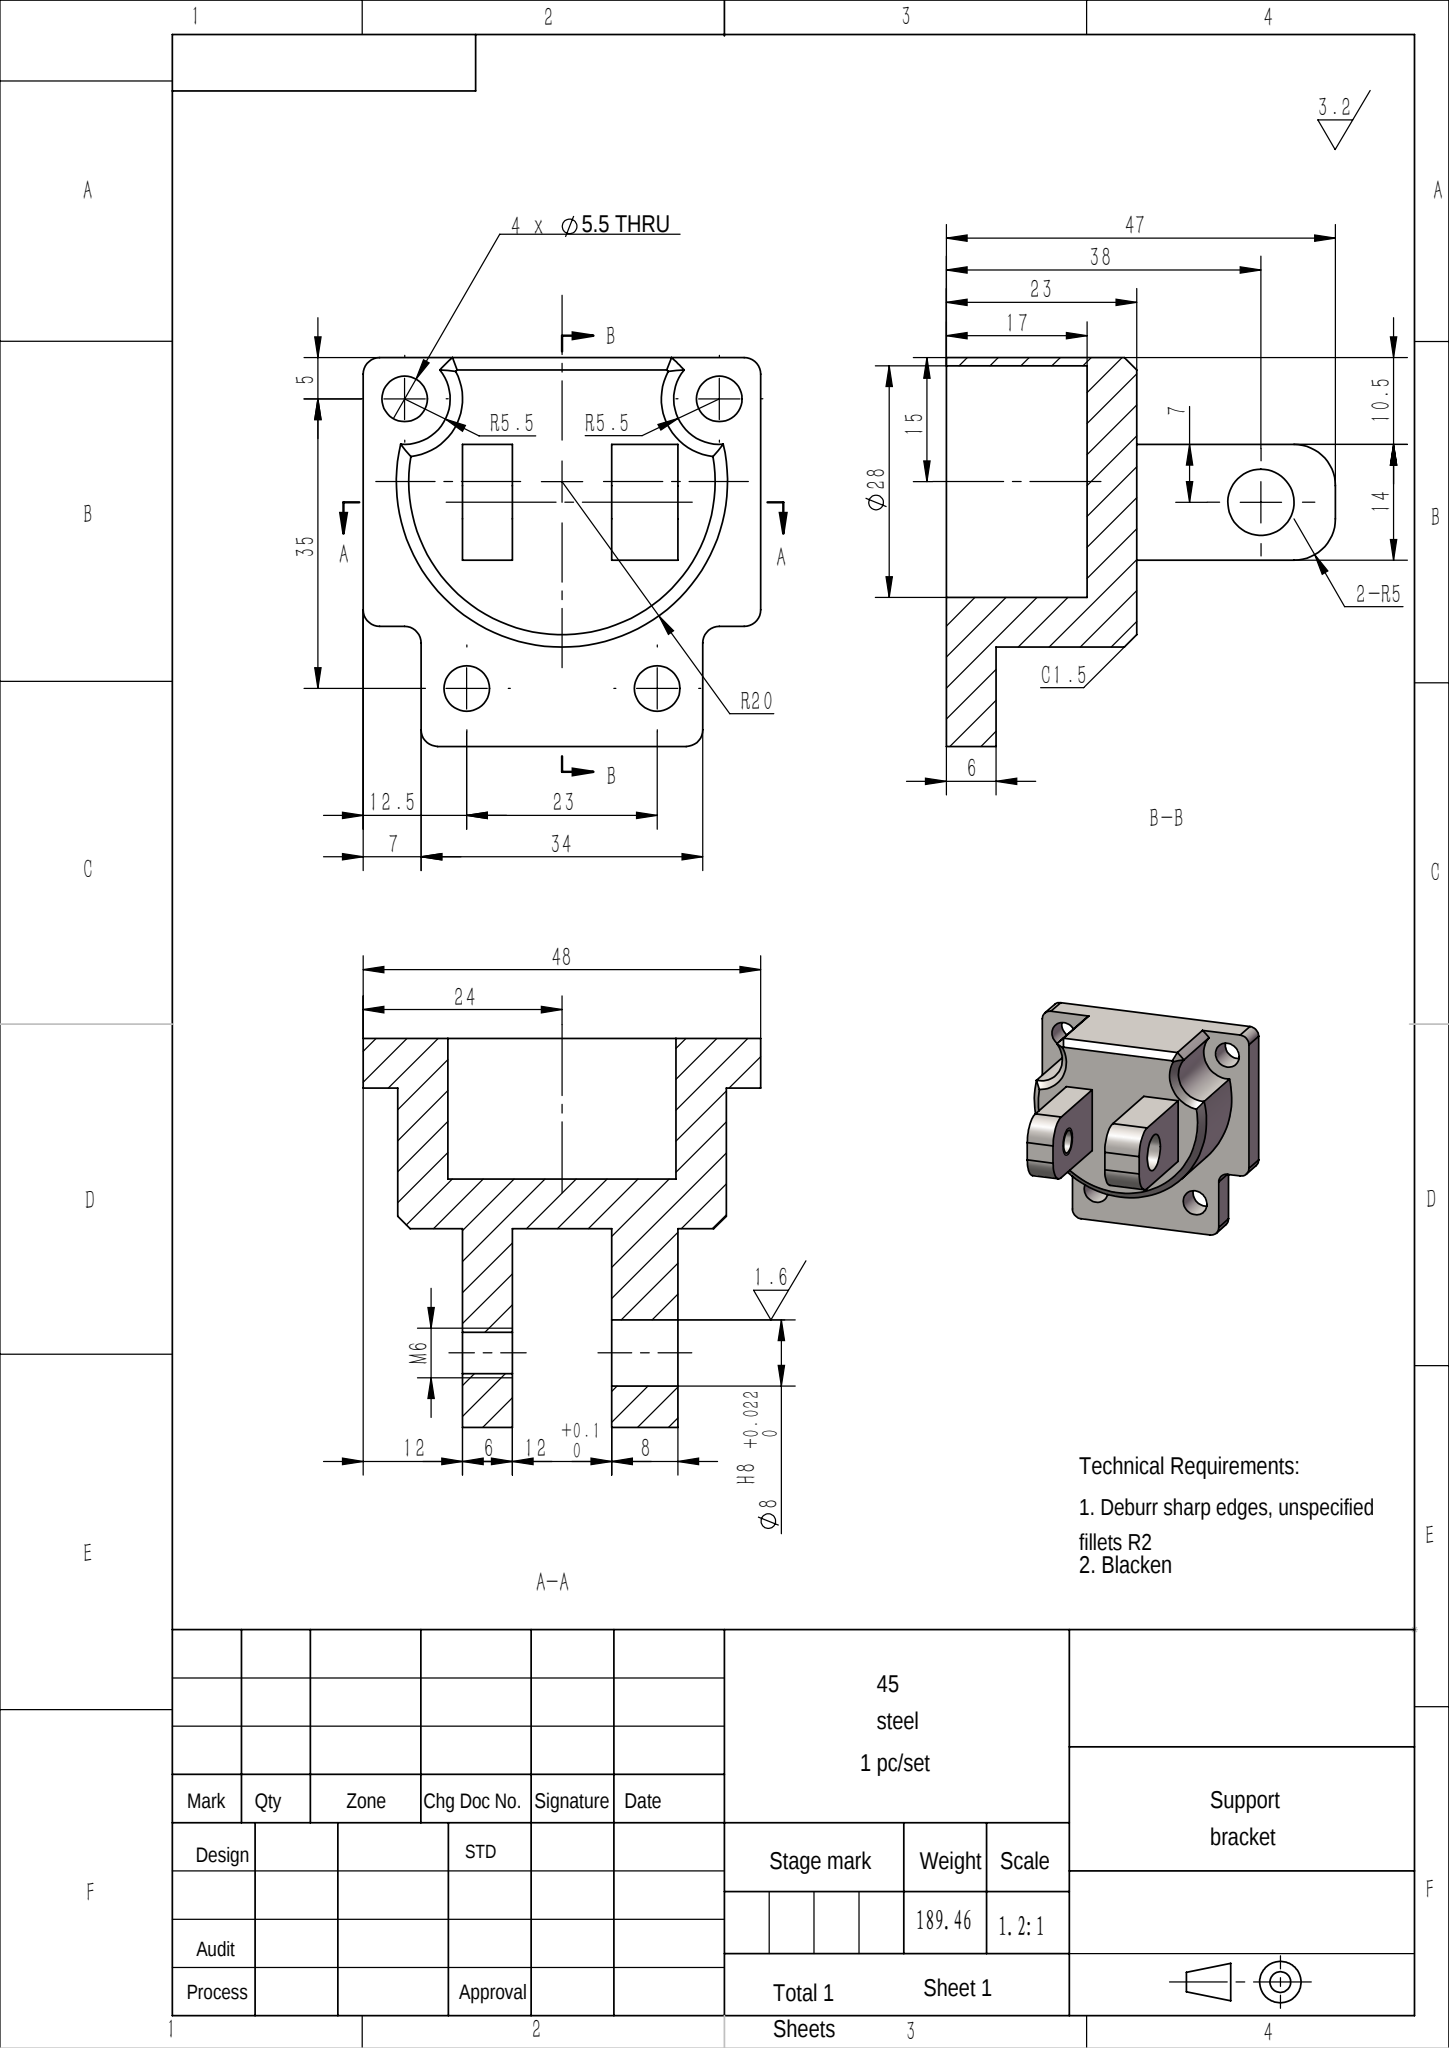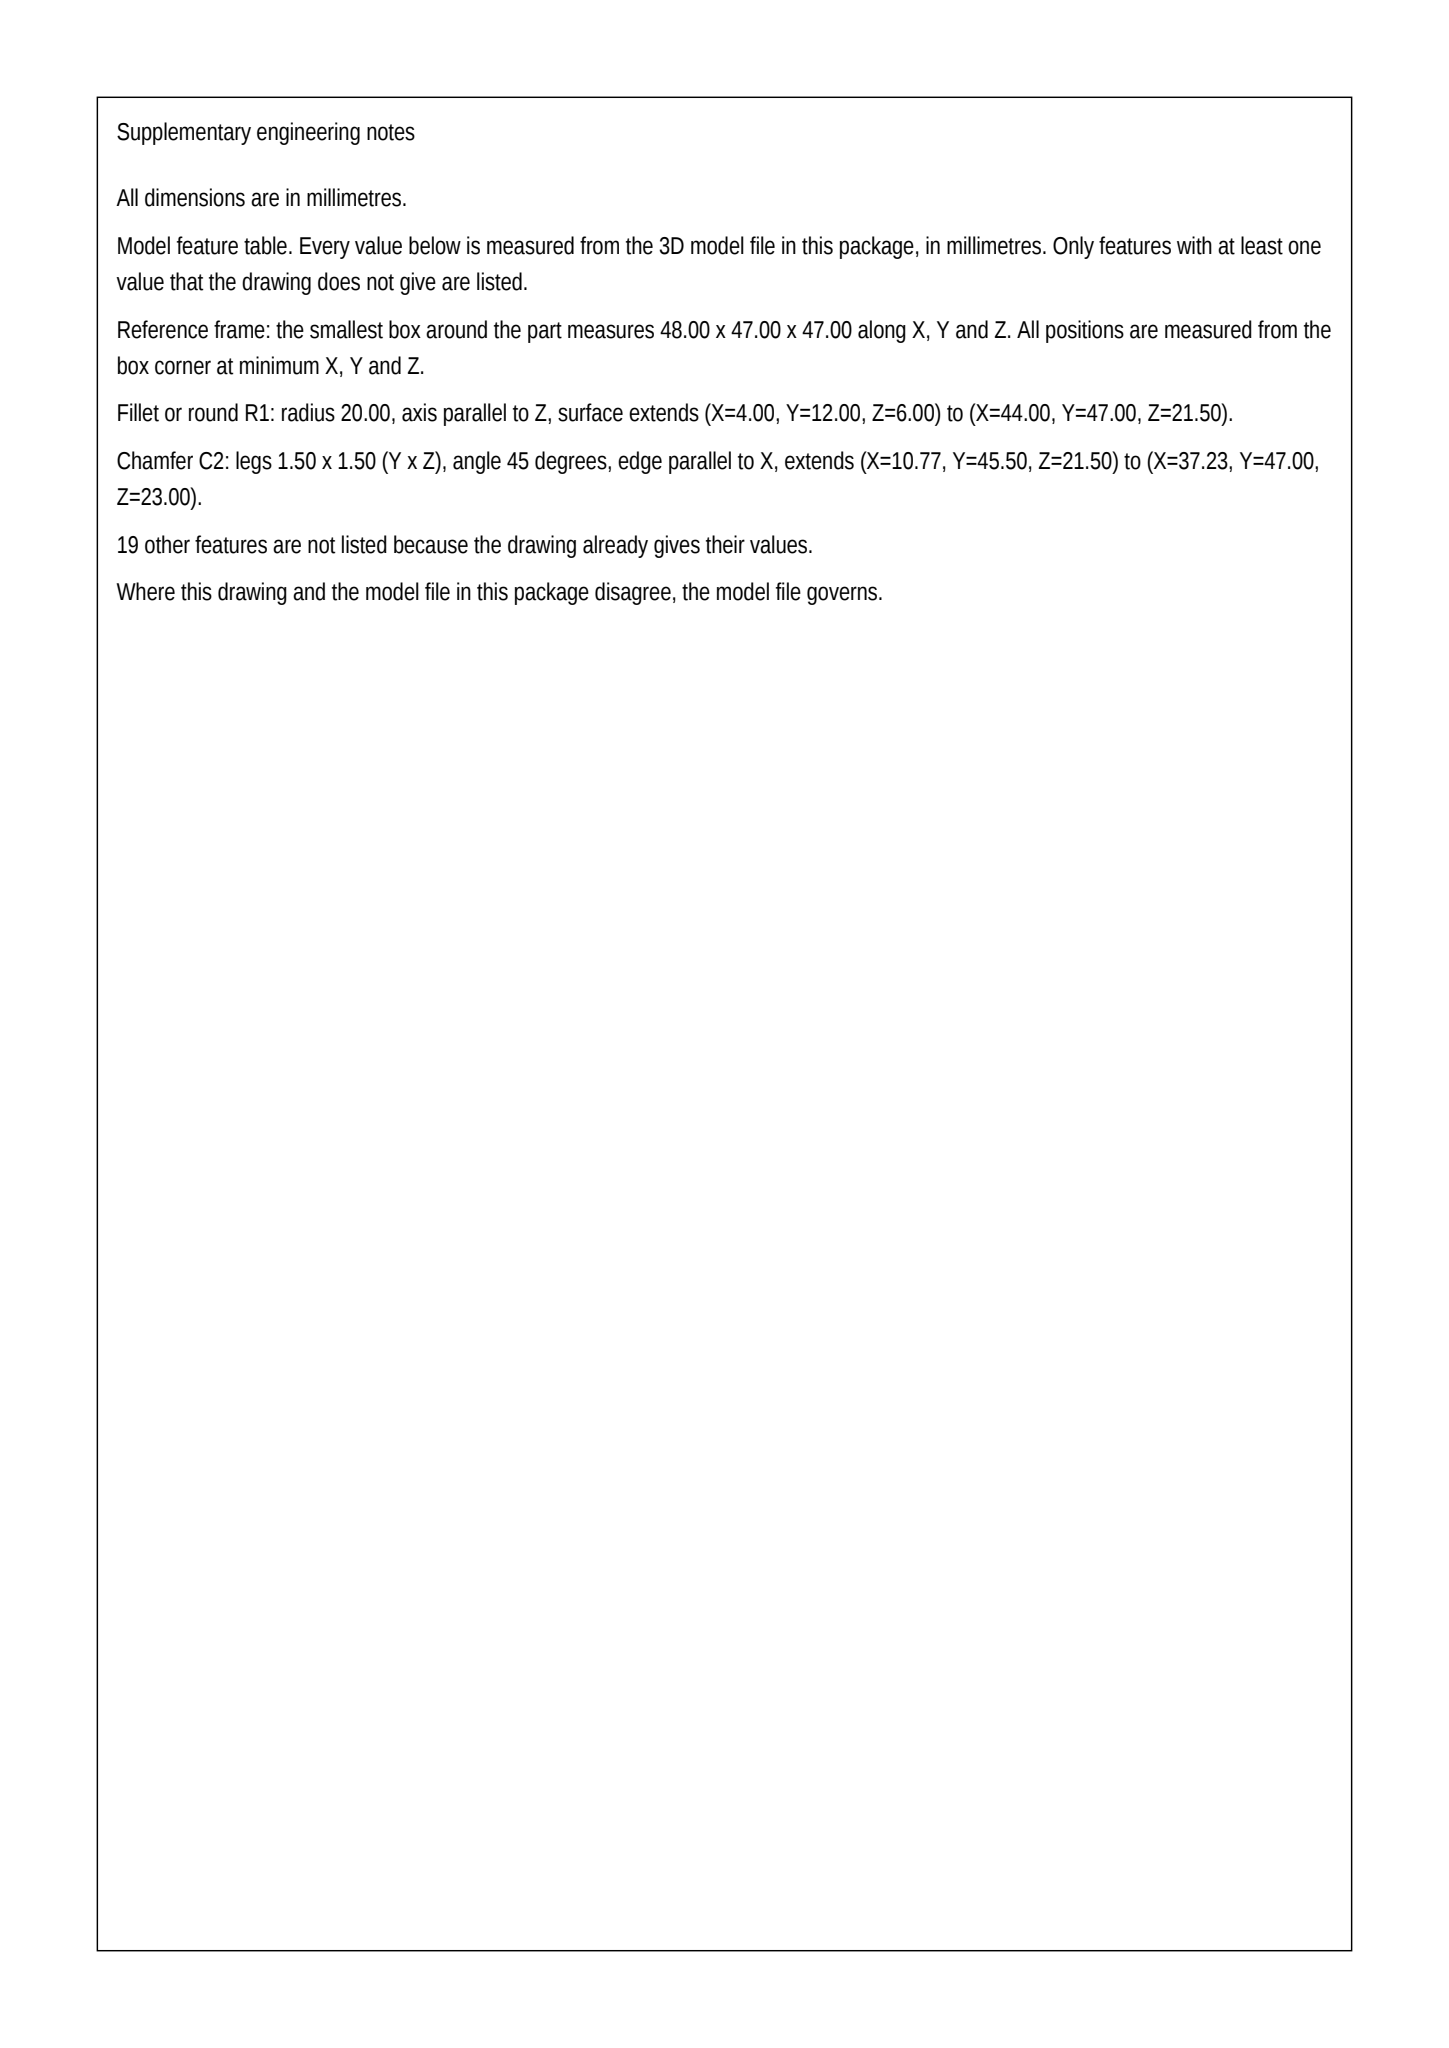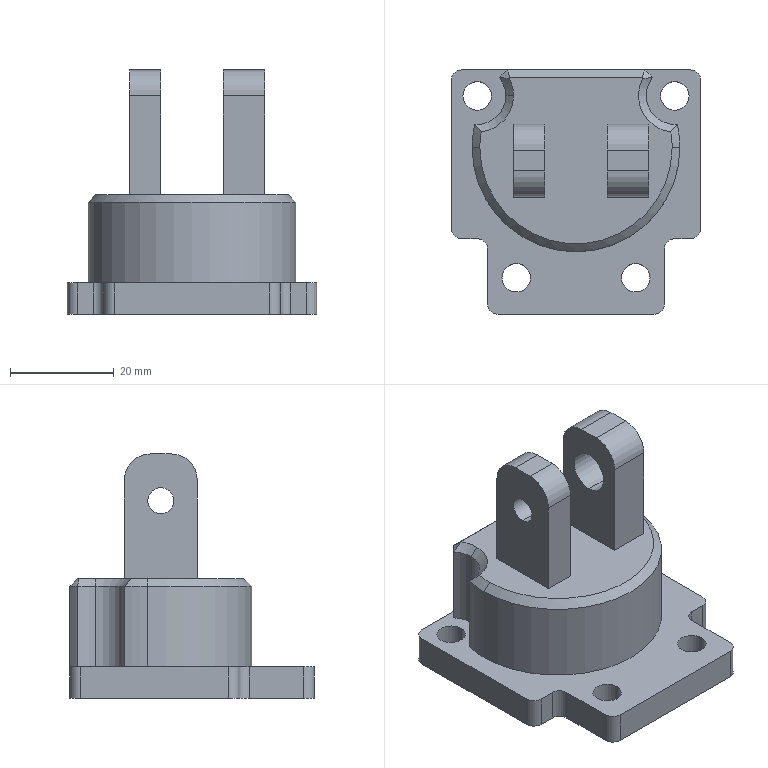Part | SolidWorks | mm | material 45 steel | 1 solid | 65 faces | box 48 x 47 x 47 mm | volume 23982 mm3 | cylinder 34 | plane 23 | cone 8 | commonest cylinder face diameters 5.5 x8 4 x8 40 x5 10 x4 11 x3 28 x2 5 x2 8 x2
build123d program:
from build123d import *

# Parameters (mm, degrees)
SKETCH1_W                     = 48
SKETCH1_H                     = 35
BOSS_EXTRUDE1_DEPTH           = 23
SKETCH2_W                     = 6
SKETCH2_H                     = 14
BOSS_EXTRUDE2_DEPTH           = 24
F_8_0_8_DIAMETER_HOLE1_D      = 8
F_8_0_8_DIAMETER_HOLE1_DEPTH  = 6
M6_TAPPED_HOLE1_D             = 5
MOVE_FACE1_BY                 = 2
SKETCH10_W                    = 34
SKETCH10_H                    = 12
BOSS_EXTRUDE3_DEPTH           = 23
MOVE_FACE2_BY                 = 2.5
MOVE_FACE2_2_BY               = 2.5
FILLET1_R                     = 5
FILLET2_R                     = 2
SKETCH11_R                    = 14
CUT_EXTRUDE1_DEPTH            = 17
SKETCH16_OUTSIDE_W            = 66.398
SKETCH16_OUTSIDE_H            = 65.398
SKETCH16_OUTSIDE_R            = 20
CUT_EXTRUDE4_DEPTH            = 17
SKETCH7_W                     = 2.75
SKETCH7_H                     = 6
M5_CLEARANCE_HOLE1_AT_2_COUNT = 2
M5_CLEARANCE_HOLE1_AT_2_PITCH = 35.795
M5_CLEARANCE_HOLE1_AT_3_COUNT = 2
M5_CLEARANCE_HOLE1_AT_3_PITCH = 46.425
M5_CLEARANCE_HOLE1_AT_4_COUNT = 2
M5_CLEARANCE_HOLE1_AT_4_PITCH = 38
SKETCH14_R                    = 5.5
CUT_EXTRUDE3_DEPTH            = 17
CHAMFER1_SIZE                 = 1.5


with BuildPart() as part:
    # Sketch1 → Boss-Extrude1 (new body)
    with BuildSketch(Plane.XY):
        Rectangle(SKETCH1_W, SKETCH1_H)
    extrude(amount=BOSS_EXTRUDE1_DEPTH)

    # Sketch2 → Boss-Extrude2 (add)
    with BuildSketch(Plane.XY.offset(23)):
        with Locations((-9, 0)):
            Rectangle(SKETCH2_W, SKETCH2_H)
        with Locations((9, 0)):
            Rectangle(SKETCH2_W, SKETCH2_H)
    extrude(amount=BOSS_EXTRUDE2_DEPTH)

    # 8.0 _8_ Diameter Hole1
    with Locations(Plane(origin=(12, 0, 0), x_dir=(0, 0, -1), z_dir=(1, 0, 0))):
        with Locations((-38, 0)):
            Hole(F_8_0_8_DIAMETER_HOLE1_D / 2, depth=F_8_0_8_DIAMETER_HOLE1_DEPTH)

    # M6 Tapped Hole1 (through all)
    with Locations(Plane(origin=(-6, 0, 0), x_dir=(0, 0, -1), z_dir=(1, 0, 0))):
        with Locations((-38, 0)):
            Hole(M6_TAPPED_HOLE1_D / 2)

    # Move Face1: a face moved outward by 2.0
    extrude(part.faces().sort_by_distance((12, 0, 29))[0], amount=MOVE_FACE1_BY, dir=(1, 0, 0))

    # Sketch10 → Boss-Extrude3 (add, through all)
    with BuildSketch(Plane.XY.offset(23)):
        with Locations((0, -23.5)):
            Rectangle(SKETCH10_W, SKETCH10_H)
    extrude(amount=-BOSS_EXTRUDE3_DEPTH)

    # Move Face2: a face moved inward by 2.5
    extrude(part.faces().sort_by_distance((20.5, -17.5, 11.5))[0], amount=MOVE_FACE2_BY, dir=(0, 1, 0), mode=Mode.SUBTRACT)

    # Move Face2 2: a face moved inward by 2.5
    extrude(part.faces().sort_by_distance((-20.5, -17.5, 11.5))[0], amount=MOVE_FACE2_2_BY, dir=(0, 1, 0), mode=Mode.SUBTRACT)

    # Fillet1
    fillet1_edges = [part.edges().sort_by_distance(p)[0] for p in [
        (-9, -7, 47),
        (-9, 7, 47),
        (10, 7, 47),
        (10, -7, 47),
    ]]
    fillet(fillet1_edges, radius=FILLET1_R)

    # Fillet2
    fillet2_edges = [part.edges().sort_by_distance(p)[0] for p in [
        (-17, -29.5, 11.5),
        (-17, -15, 11.5),
        (17, -15, 11.5),
        (17, -29.5, 11.5),
        (24, -15, 11.5),
        (-24, -15, 11.5),
        (-24, 17.5, 11.5),
        (24, 17.5, 11.5),
    ]]
    fillet(fillet2_edges, radius=FILLET2_R)

    # Sketch11 → Cut-Extrude1 (cut)
    with BuildSketch(Plane(origin=(0, 0, 0), x_dir=(-1, 0, 0), z_dir=(0, 0, -1))):
        with Locations((0, 2.5)):
            Circle(SKETCH11_R)
    extrude(amount=-CUT_EXTRUDE1_DEPTH, mode=Mode.SUBTRACT)

    # Sketch16 outside → Cut-Extrude4 (cut)
    with BuildSketch(Plane.XY.offset(23)):
        with Locations((0, -6)):
            Rectangle(SKETCH16_OUTSIDE_W, SKETCH16_OUTSIDE_H)
        with Locations((0, 2.5)):
            Circle(SKETCH16_OUTSIDE_R, mode=Mode.SUBTRACT)
    extrude(amount=-CUT_EXTRUDE4_DEPTH, mode=Mode.SUBTRACT)

    # Sketch7 → M5 Clearance Hole1 (revolve, cut)
    with BuildSketch(Plane(origin=(-19, 12.5, 6), x_dir=(0, -1, 0), z_dir=(1, 0, 0))):
        with Locations((1.375, 3)):
            Rectangle(SKETCH7_W, SKETCH7_H)
    m5_clearance_hole1 = revolve(axis=Axis((-19, 12.5, 12.35), (0, 0, -1)), mode=Mode.SUBTRACT)

    # M5 Clearance Hole1 at 2: M5 Clearance Hole1 ×2
    with Locations(*[Vector(0.2095, -0.9778, 0) * (i * M5_CLEARANCE_HOLE1_AT_2_PITCH) for i in range(1, M5_CLEARANCE_HOLE1_AT_2_COUNT)]):
        add(m5_clearance_hole1, mode=Mode.SUBTRACT)

    # M5 Clearance Hole1 at 3: M5 Clearance Hole1 ×2
    with Locations(*[Vector(0.657, -0.7539, 0) * (i * M5_CLEARANCE_HOLE1_AT_3_PITCH) for i in range(1, M5_CLEARANCE_HOLE1_AT_3_COUNT)]):
        add(m5_clearance_hole1, mode=Mode.SUBTRACT)

    # M5 Clearance Hole1 at 4: M5 Clearance Hole1 ×2
    with Locations(*[(i * M5_CLEARANCE_HOLE1_AT_4_PITCH, 0, 0) for i in range(1, M5_CLEARANCE_HOLE1_AT_4_COUNT)]):
        add(m5_clearance_hole1, mode=Mode.SUBTRACT)

    # Sketch14 → Cut-Extrude3 (cut)
    with BuildSketch(Plane.XY.offset(23)):
        with Locations((-19, 12.5)):
            Circle(SKETCH14_R)
        with Locations((19, 12.5)):
            Circle(SKETCH14_R)
    extrude(amount=-CUT_EXTRUDE3_DEPTH, mode=Mode.SUBTRACT)

    # Chamfer1
    chamfer1_edges = [part.edges().sort_by_distance(p)[0] for p in [
        (0, 17.5, 23),
        (-14.013, 16.77, 23),
        (0, -17.5, 23),
        (14.013, 16.77, 23),
        (-14.133, 9.938, 23),
        (14.133, 9.938, 23),
    ]]
    chamfer(chamfer1_edges, length=CHAMFER1_SIZE)


solid = part.part